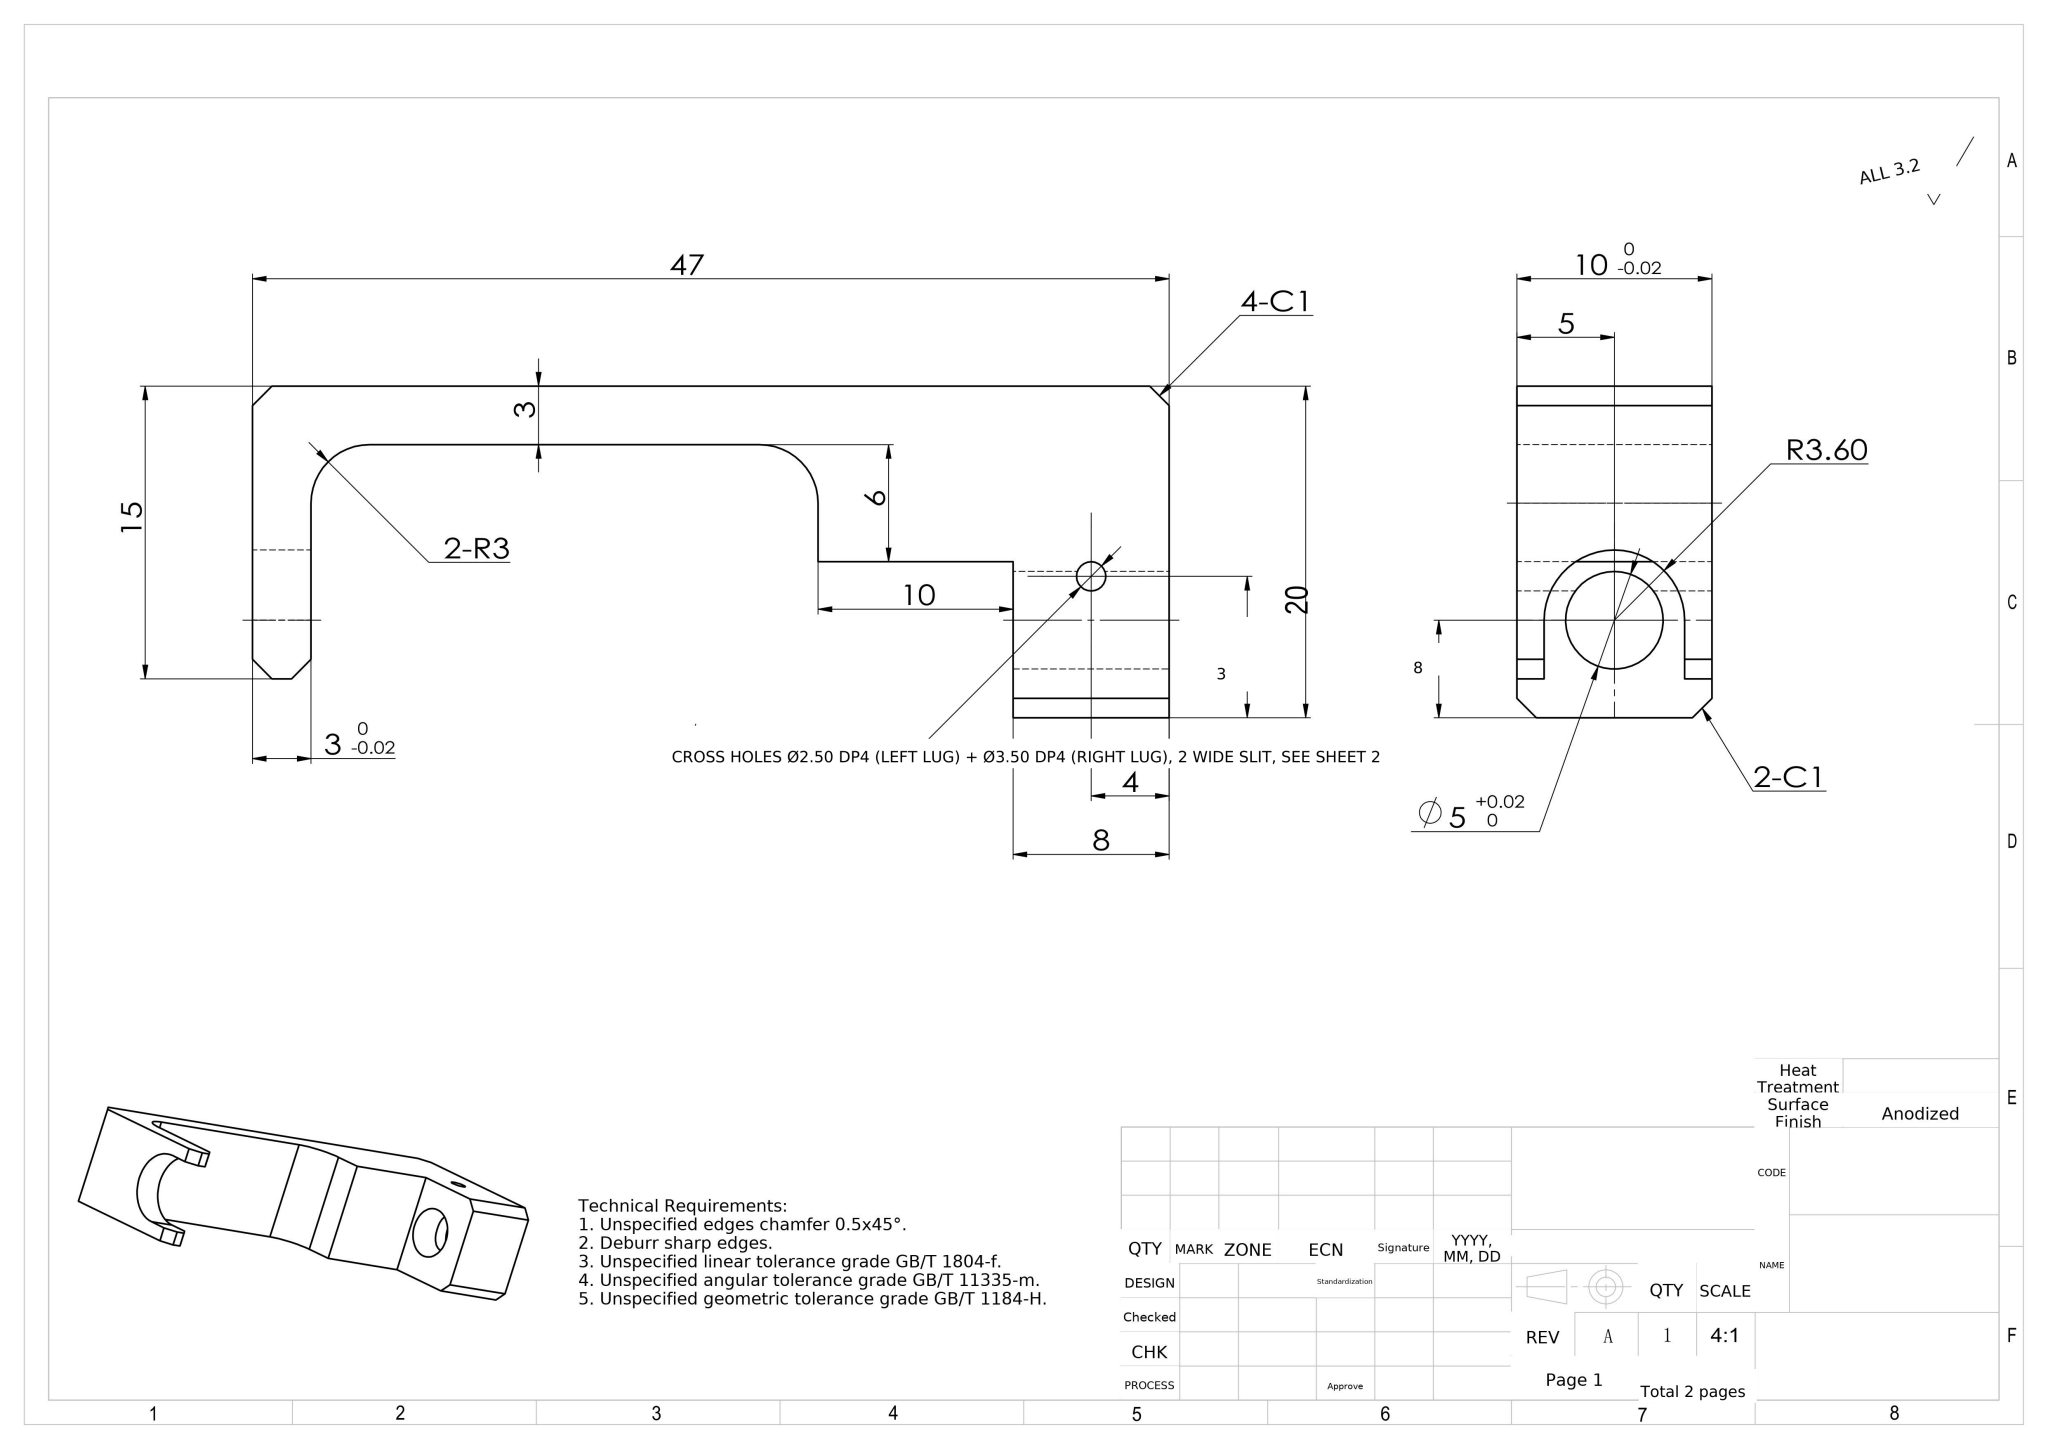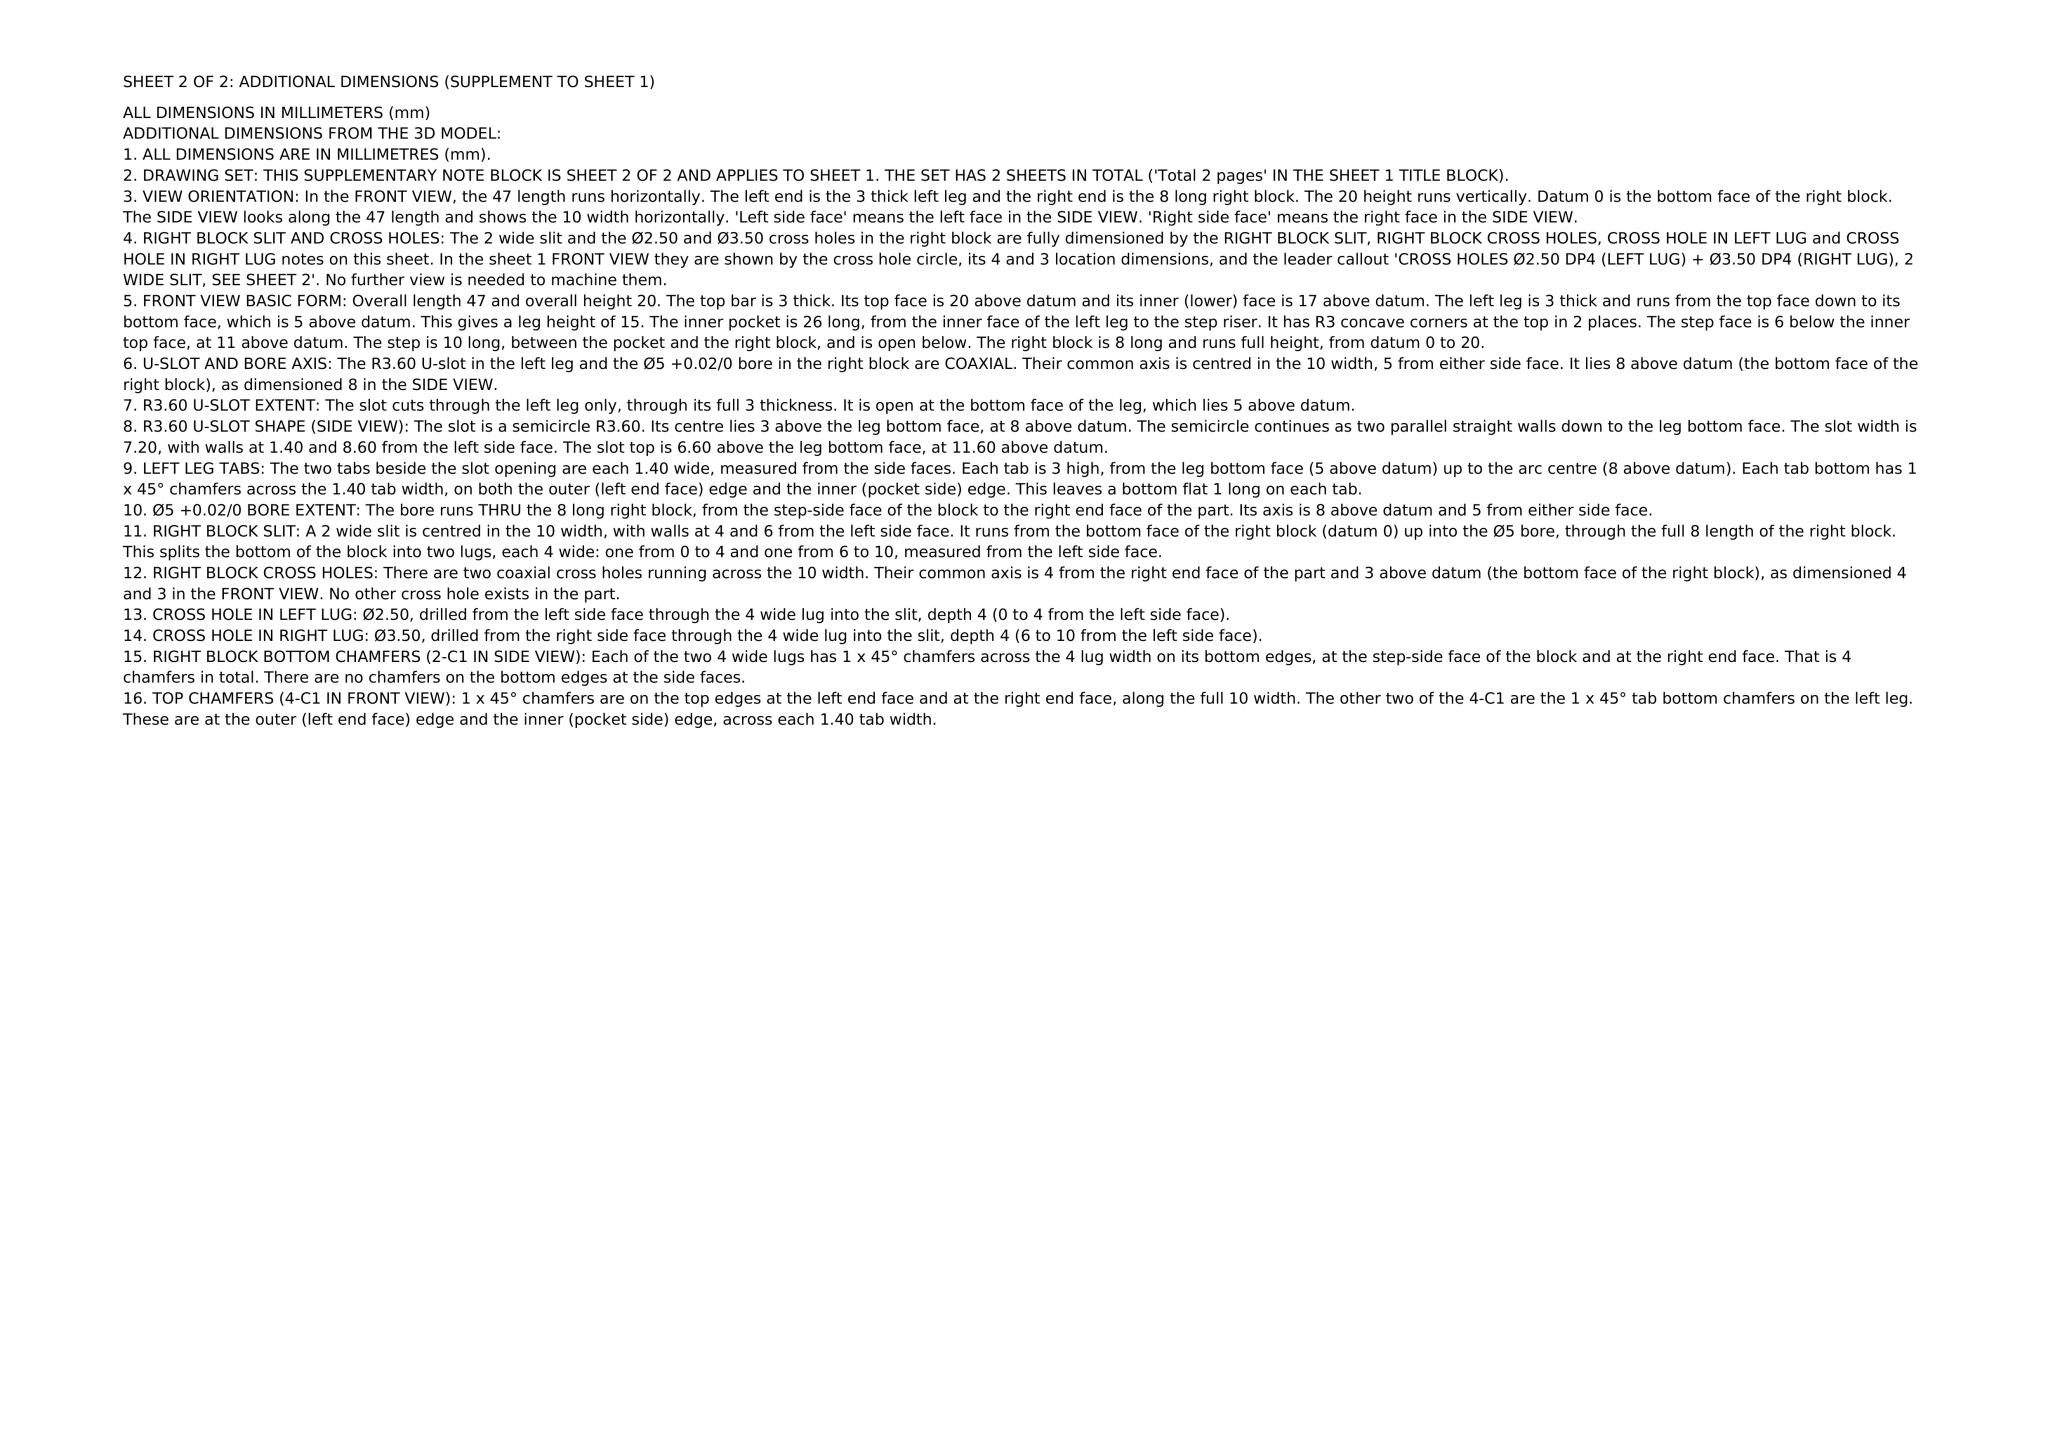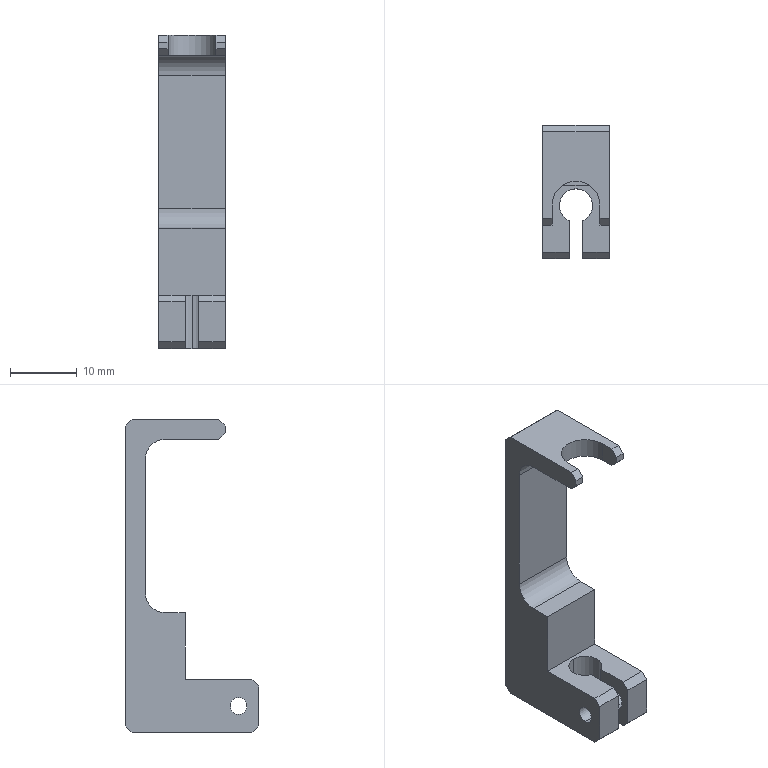Part | NX | mm | 1 solid | 37 faces | box 10 x 20 x 47 mm | volume 3318 mm3 | plane 28 | cylinder 9 | commonest cylinder face diameters 3.5 x2 2.5 x2 5 x2 6 x2 7.2 x1